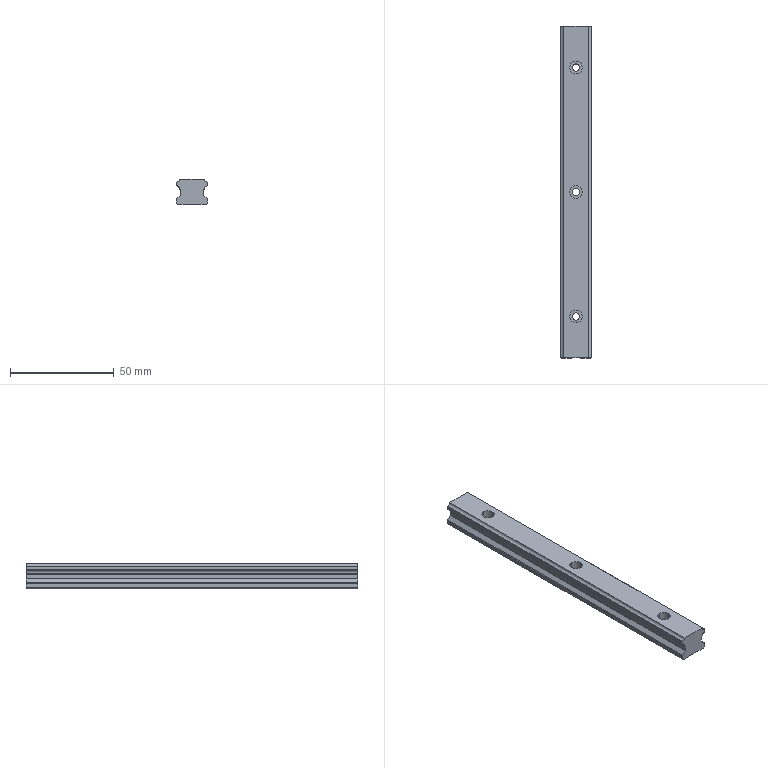Component | SolidWorks | CCDJSBufferChainBlanking-Z-Axis-LinearGuide-EGH15CA1R160-2_CCDJSBufferChainBlanking-Lifting-LinearGuide-EGR15R160-1 | 1 solid | 52 faces | box 15 x 160 x 12.43 mm | volume 25394 mm3 | cylinder 29 | plane 23 | commonest cylinder face diameters 0.6 x10 6 x6 3.5 x6 3 x5 1 x2 | material AISI 304
build123d program:
from build123d import *

# Parameters (mm, degrees)
BOSS_EXTRUDE1_DEPTH                             = 80
M3_HEX_SOCKET_HEAD_CAP_SCREW_CBORE1_D           = 3.5
M3_HEX_SOCKET_HEAD_CAP_SCREW_CBORE1_CBORE_D     = 6
M3_HEX_SOCKET_HEAD_CAP_SCREW_CBORE1_CBORE_DEPTH = 4.5
LPATTERN1_COUNT                                 = 3
LPATTERN1_PITCH                                 = 60
CUT_EXTRUDE1_START                              = -80
SKETCH1_W                                       = 16
SKETCH1_H                                       = 1.37
CUT_EXTRUDE1_DEPTH                              = 160


with BuildPart() as part:
    # Sketch1_2 → Boss-Extrude1 (new, symmetric)
    with BuildSketch(Plane.XY):
        with BuildLine():
            Line((6.029, 7.336), (5.588, 6.894))
            ThreePointArc((5.588, 6.894), (5.523, 6.797), (5.5, 6.682))
            Line((5.5, 6.682), (5.5, 4.524))
            ThreePointArc((5.5, 4.524), (5.523, 4.409), (5.588, 4.312))
            Line((5.588, 4.312), (7.354, 2.546))
            ThreePointArc((7.354, 2.546), (7.462, 2.384), (7.5, 2.193))
            Line((7.5, 2.193), (7.5, 0.4))
            Line((7.5, 0.4), (6.8, -0.3))
            Line((6.8, -0.3), (2.35, -0.3))
            Line((2.35, -0.3), (2.05, 0))
            Line((2.05, 0), (-2.05, 0))
            Line((-2.05, 0), (-2.35, -0.3))
            Line((-2.35, -0.3), (-6.8, -0.3))
            Line((-6.8, -0.3), (-7.5, 0.4))
            Line((-7.5, 0.4), (-7.5, 2.193))
            ThreePointArc((-7.5, 2.193), (-7.462, 2.384), (-7.354, 2.546))
            Line((-7.354, 2.546), (-5.588, 4.312))
            ThreePointArc((-5.588, 4.312), (-5.523, 4.409), (-5.5, 4.524))
            Line((-5.5, 4.524), (-5.5, 6.682))
            ThreePointArc((-5.5, 6.682), (-5.523, 6.797), (-5.588, 6.894))
            Line((-5.588, 6.894), (-6.029, 7.336))
            ThreePointArc((-6.029, 7.336), (-6.419, 8.38), (-7.422, 8.867))
            ThreePointArc((-7.422, 8.867), (-7.48, 8.961), (-7.5, 9.069))
            Line((-7.5, 9.069), (-7.5, 10.531))
            ThreePointArc((-7.5, 10.531), (-7.48, 10.639), (-7.422, 10.733))
            ThreePointArc((-7.422, 10.733), (-6.468, 11.168), (-6.033, 12.122))
            ThreePointArc((-6.033, 12.122), (-5.939, 12.18), (-5.831, 12.2))
            Line((-5.831, 12.2), (5.831, 12.2))
            ThreePointArc((5.831, 12.2), (5.939, 12.18), (6.033, 12.122))
            ThreePointArc((6.033, 12.122), (6.468, 11.168), (7.422, 10.733))
            ThreePointArc((7.422, 10.733), (7.48, 10.639), (7.5, 10.531))
            Line((7.5, 10.531), (7.5, 9.069))
            ThreePointArc((7.5, 9.069), (7.48, 8.961), (7.422, 8.867))
            ThreePointArc((7.422, 8.867), (6.419, 8.38), (6.029, 7.336))
        make_face()
    extrude(amount=BOSS_EXTRUDE1_DEPTH, both=True)

    # M3 Hex Socket Head Cap Screw CBORE1 (through all)
    with Locations(Plane(origin=(0, 12.2, 0), x_dir=(1, 0, 0), z_dir=(0, 1, 0))):
        with Locations((0, -60)):
            m3_hex_socket_head_cap_screw_cbore1 = CounterBoreHole(M3_HEX_SOCKET_HEAD_CAP_SCREW_CBORE1_D / 2, M3_HEX_SOCKET_HEAD_CAP_SCREW_CBORE1_CBORE_D / 2, M3_HEX_SOCKET_HEAD_CAP_SCREW_CBORE1_CBORE_DEPTH)

    # LPattern1: M3 Hex Socket Head Cap Screw CBORE1 ×3
    with Locations(*[(0, 0, -i * LPATTERN1_PITCH) for i in range(1, LPATTERN1_COUNT)]):
        add(m3_hex_socket_head_cap_screw_cbore1, mode=Mode.SUBTRACT)

    # Sketch1 → Cut-Extrude1 (cut)
    with BuildSketch(Plane.XY.offset(CUT_EXTRUDE1_START)):
        with Locations((0, 12.815)):
            Rectangle(SKETCH1_W, SKETCH1_H)
    extrude(amount=CUT_EXTRUDE1_DEPTH, mode=Mode.SUBTRACT)


solid = part.part

# Placed as in the assembly
solid = solid.moved(Location((-158.9, 428.464, -92.27), (90, 0, 0)))